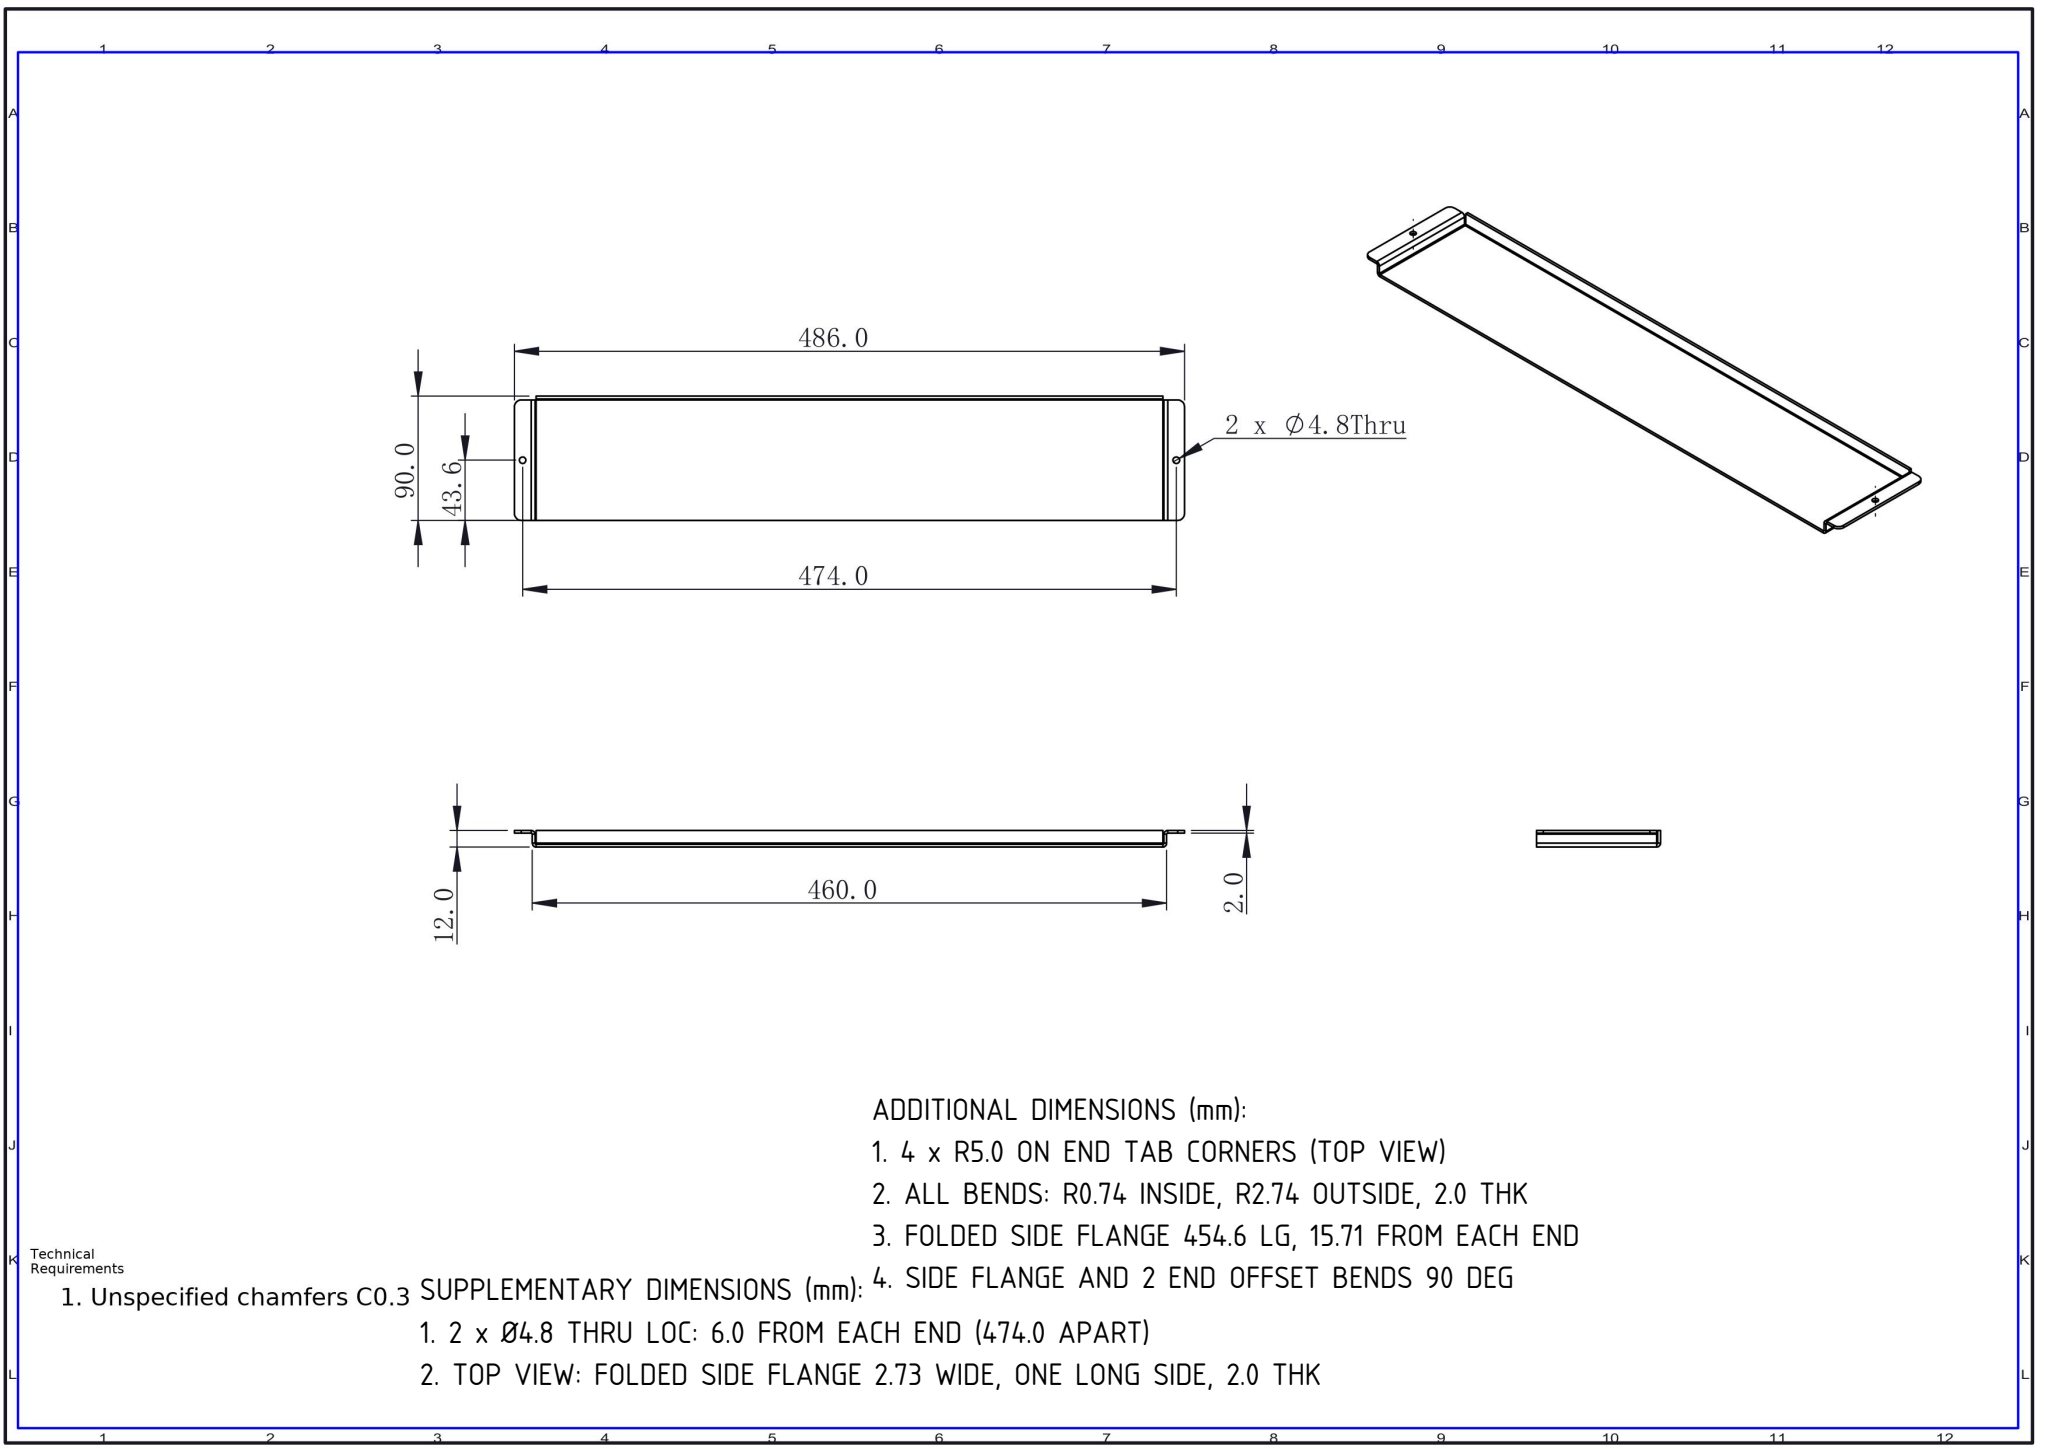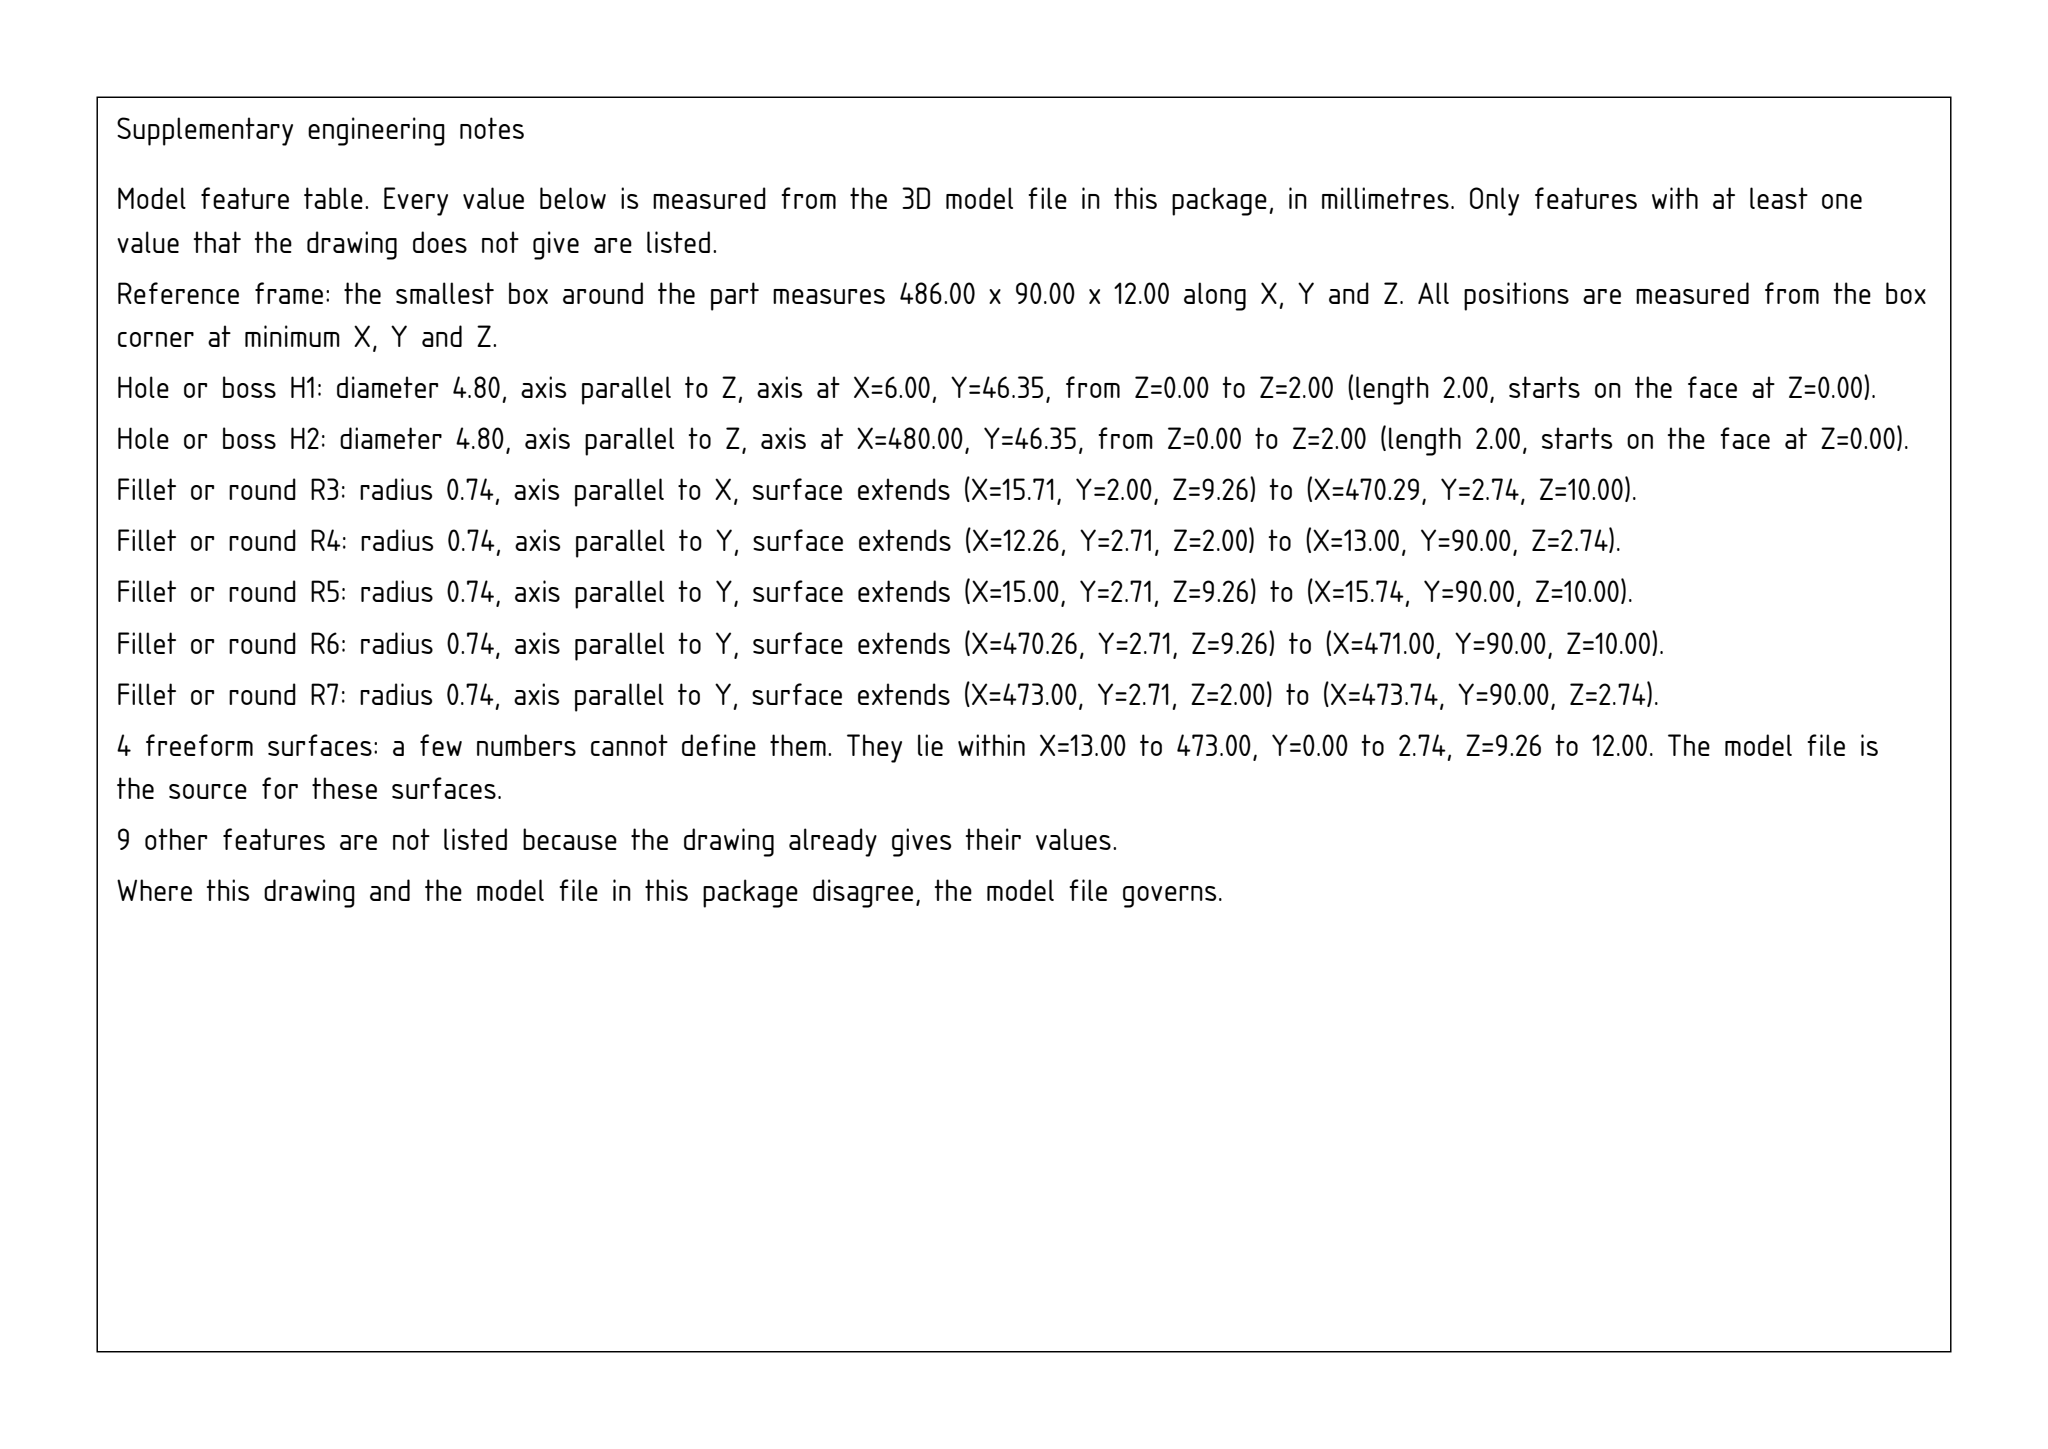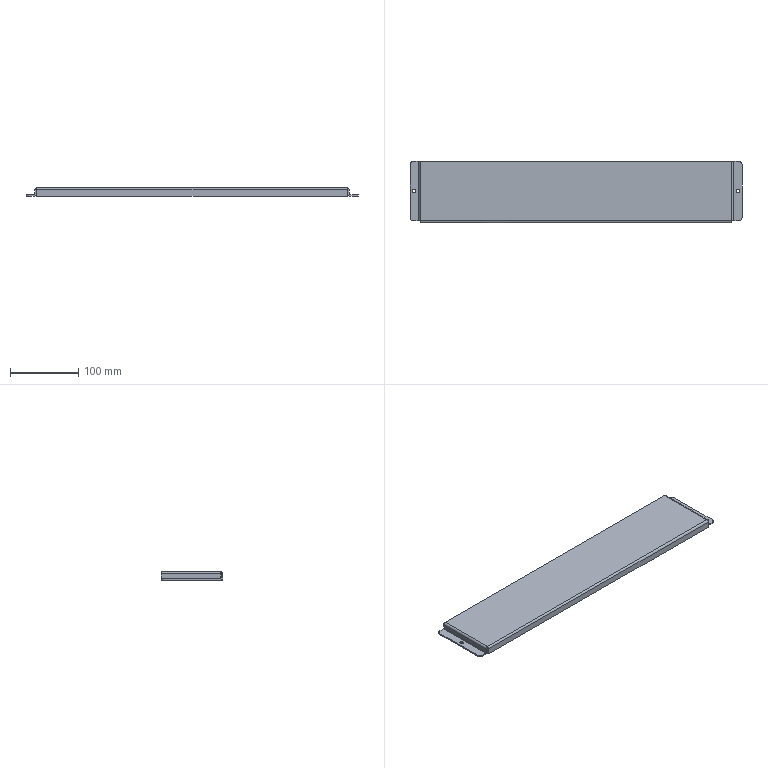Part | SolidWorks | mm | 1 solid | 54 faces | box 486 x 90 x 12 mm | volume 98580 mm3 | plane 32 | cylinder 18 | spline 4 | commonest cylinder face diameters 5.473 x5 1.473 x5 4.8 x4 10 x4